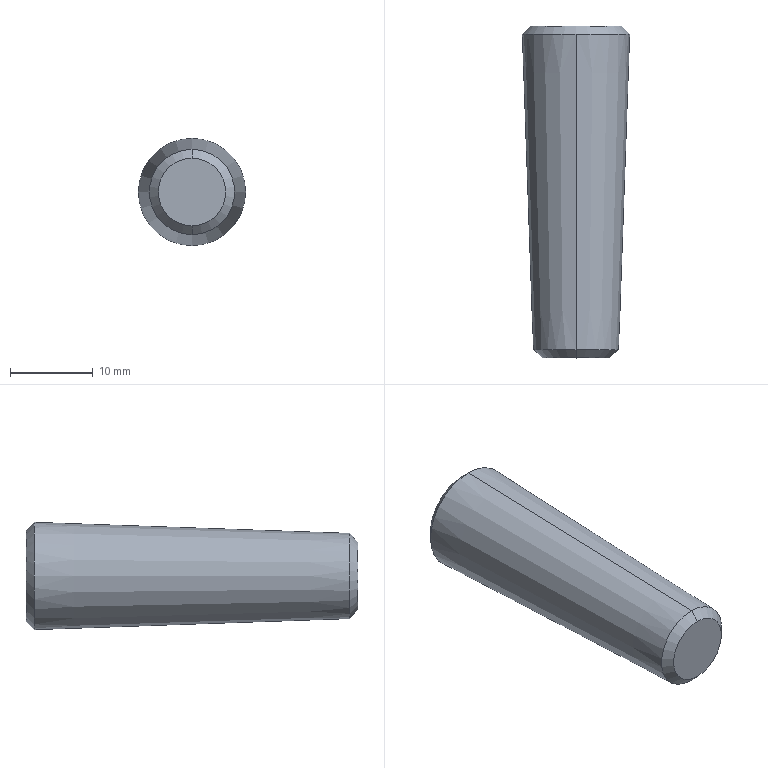Component | SolidWorks | TaperPin-1 | 1 solid | 8 faces | box 12.93 x 40 x 12.93 mm | volume 4216 mm3 | cone 6 | plane 2
build123d program:
from build123d import *
from OCP.BRepFilletAPI import BRepFilletAPI_MakeChamfer

# Parameters (mm, degrees)
CHAMFER1_SIZE    = 1
CHAMFER1_SIZE2   = 1.037
CHAMFER1_SIZE2_2 = 0.9668


with BuildPart() as part:
    # Sketch1 → Revolve4 (revolve)
    with BuildSketch(Plane.XY, mode=Mode.PRIVATE) as revolve4_sk:
        Polygon((6.5, 40), (5.103, 0), (0, 0), (0, 40), align=None)
    revolve(revolve4_sk.sketch.rotate(Axis((0, 0, 0), (0, 1, 0)), 90), axis=Axis((0, 0, 0), (0, 1, 0)))

    # Chamfer1: one chamfer whose edges measure the first distance from different faces: ONE call of the kernel's chamfer builder (chamfer() names one face for all edges)
    chamfer1_edges_1 = [part.edges().sort_by_distance(p)[0] for p in [
        (0, 0, 5.103),
    ]]
    chamfer1_side_1 = [part.faces().sort_by_distance(p)[0] for p in [
        (0, 20, 5.802),
    ]]
    chamfer1_edges_2 = [part.edges().sort_by_distance(p)[0] for p in [
        (0, 40, 6.5),
    ]]
    chamfer1_side_2 = [part.faces().sort_by_distance(p)[0] for p in [
        (0, 40, 0),
    ]]
    chamfer1 = BRepFilletAPI_MakeChamfer(part.part.solid().wrapped)
    for e in chamfer1_edges_1:
        chamfer1.Add(CHAMFER1_SIZE, CHAMFER1_SIZE2, e.wrapped, chamfer1_side_1[0].wrapped)  # the first distance lies on this face
    for e in chamfer1_edges_2:
        chamfer1.Add(CHAMFER1_SIZE, CHAMFER1_SIZE2_2, e.wrapped, chamfer1_side_2[0].wrapped)  # the first distance lies on this face
    add(Compound.cast(chamfer1.Shape()), mode=Mode.REPLACE)


solid = part.part

# Placed as in the assembly
solid = solid.moved(Location((726.83, 1259.341, 1507.217), (0, 0, 0)))
STEP:
#1=COLOUR_RGB('',0.7922,0.8196,0.9333);
#2=FILL_AREA_STYLE_COLOUR('',#1);
#3=FILL_AREA_STYLE('',(#2));
#4=SURFACE_STYLE_FILL_AREA(#3);
#5=SURFACE_SIDE_STYLE('',(#4));
#6=SURFACE_STYLE_USAGE(.BOTH.,#5);
#7=PRESENTATION_STYLE_ASSIGNMENT((#6));
#8=CARTESIAN_POINT('',(28.615,51.155,59.556));
#9=VERTEX_POINT('',#8);
#10=CARTESIAN_POINT('',(28.615,51.155,59.123));
#11=VERTEX_POINT('',#10);
#12=CARTESIAN_POINT('',(28.615,51.155,59.339));
#13=DIRECTION('',(0.,1.,0.));
#14=DIRECTION('',(0.,0.,-1.));
#15=AXIS2_PLACEMENT_3D('',#12,#13,#14);
#16=CIRCLE('',#15,0.2165);
#17=EDGE_CURVE('',#9,#11,#16,.T.);
#18=ORIENTED_EDGE('',*,*,#17,.F.);
#19=CARTESIAN_POINT('',(28.615,51.117,59.594));
#20=VERTEX_POINT('',#19);
#21=CARTESIAN_POINT('',(28.615,51.117,59.594));
#22=DIRECTION('',(0.,-0.7071,0.7071));
#23=VECTOR('',#22,39.37);
#24=LINE('',#21,#23);
#25=EDGE_CURVE('',#9,#20,#24,.T.);
#26=ORIENTED_EDGE('',*,*,#25,.T.);
#27=CARTESIAN_POINT('',(28.615,51.117,59.085));
#28=VERTEX_POINT('',#27);
#29=CARTESIAN_POINT('',(28.615,51.117,59.339));
#30=DIRECTION('',(0.,-1.,0.));
#31=DIRECTION('',(0.,0.,-1.));
#32=AXIS2_PLACEMENT_3D('',#29,#30,#31);
#33=CIRCLE('',#32,0.2546);
#34=EDGE_CURVE('',#28,#20,#33,.T.);
#35=ORIENTED_EDGE('',*,*,#34,.F.);
#36=CARTESIAN_POINT('',(28.615,51.117,59.085));
#37=DIRECTION('',(0.,-0.7071,-0.7071));
#38=VECTOR('',#37,39.37);
#39=LINE('',#36,#38);
#40=EDGE_CURVE('',#11,#28,#39,.T.);
#41=ORIENTED_EDGE('',*,*,#40,.F.);
#42=EDGE_LOOP('',(#18,#26,#35,#41));
#43=FACE_OUTER_BOUND('',#42,.T.);
#44=CARTESIAN_POINT('',(28.615,51.117,59.339));
#45=DIRECTION('',(0.,-1.,0.));
#46=DIRECTION('',(0.,0.,-1.));
#47=AXIS2_PLACEMENT_3D('',#44,#45,#46);
#48=CONICAL_SURFACE('',#47,0.2546,0.7854);
#49=ADVANCED_FACE('',(#43),#48,.T.);
#50=CARTESIAN_POINT('',(28.615,49.58,59.179));
#51=VERTEX_POINT('',#50);
#52=CARTESIAN_POINT('',(28.615,49.58,59.499));
#53=VERTEX_POINT('',#52);
#54=CARTESIAN_POINT('',(28.615,49.58,59.339));
#55=DIRECTION('',(0.,-1.,0.));
#56=DIRECTION('',(0.,0.,-1.));
#57=AXIS2_PLACEMENT_3D('',#54,#55,#56);
#58=CIRCLE('',#57,0.1601);
#59=EDGE_CURVE('',#51,#53,#58,.T.);
#60=ORIENTED_EDGE('',*,*,#59,.F.);
#61=CARTESIAN_POINT('',(28.615,49.62,59.137));
#62=VERTEX_POINT('',#61);
#63=CARTESIAN_POINT('',(28.615,49.58,59.179));
#64=DIRECTION('',(0.,0.682,-0.7314));
#65=VECTOR('',#64,39.37);
#66=LINE('',#63,#65);
#67=EDGE_CURVE('',#51,#62,#66,.T.);
#68=ORIENTED_EDGE('',*,*,#67,.T.);
#69=CARTESIAN_POINT('',(28.615,49.62,59.542));
#70=VERTEX_POINT('',#69);
#71=CARTESIAN_POINT('',(28.615,49.62,59.339));
#72=DIRECTION('',(0.,1.,0.));
#73=DIRECTION('',(0.,0.,1.));
#74=AXIS2_PLACEMENT_3D('',#71,#72,#73);
#75=CIRCLE('',#74,0.2023);
#76=EDGE_CURVE('',#70,#62,#75,.T.);
#77=ORIENTED_EDGE('',*,*,#76,.F.);
#78=CARTESIAN_POINT('',(28.615,49.58,59.499));
#79=DIRECTION('',(0.,0.682,0.7314));
#80=VECTOR('',#79,39.37);
#81=LINE('',#78,#80);
#82=EDGE_CURVE('',#53,#70,#81,.T.);
#83=ORIENTED_EDGE('',*,*,#82,.F.);
#84=EDGE_LOOP('',(#60,#68,#77,#83));
#85=FACE_OUTER_BOUND('',#84,.T.);
#86=CARTESIAN_POINT('',(28.615,49.58,59.339));
#87=DIRECTION('',(0.,1.,0.));
#88=DIRECTION('',(0.,0.,1.));
#89=AXIS2_PLACEMENT_3D('',#86,#87,#88);
#90=CONICAL_SURFACE('',#89,0.1601,0.8203);
#91=ADVANCED_FACE('',(#85),#90,.T.);
#92=ORIENTED_EDGE('',*,*,#76,.T.);
#93=CARTESIAN_POINT('',(28.615,51.155,59.083));
#94=DIRECTION('',(0.,0.9994,-0.0349));
#95=VECTOR('',#94,39.37);
#96=LINE('',#93,#95);
#97=EDGE_CURVE('',#62,#28,#96,.T.);
#98=ORIENTED_EDGE('',*,*,#97,.T.);
#99=ORIENTED_EDGE('',*,*,#34,.T.);
#100=CARTESIAN_POINT('',(28.615,51.155,59.595));
#101=DIRECTION('',(0.,0.9994,0.0349));
#102=VECTOR('',#101,39.37);
#103=LINE('',#100,#102);
#104=EDGE_CURVE('',#70,#20,#103,.T.);
#105=ORIENTED_EDGE('',*,*,#104,.F.);
#106=EDGE_LOOP('',(#92,#98,#99,#105));
#107=FACE_OUTER_BOUND('',#106,.T.);
#108=CARTESIAN_POINT('',(28.615,51.155,59.339));
#109=DIRECTION('',(0.,1.,0.));
#110=DIRECTION('',(0.,0.,1.));
#111=AXIS2_PLACEMENT_3D('',#108,#109,#110);
#112=CONICAL_SURFACE('',#111,0.2559,0.03491);
#113=ADVANCED_FACE('',(#107),#112,.T.);
#114=ORIENTED_EDGE('',*,*,#97,.F.);
#115=CARTESIAN_POINT('',(28.615,49.62,59.339));
#116=DIRECTION('',(0.,1.,0.));
#117=DIRECTION('',(0.,0.,1.));
#118=AXIS2_PLACEMENT_3D('',#115,#116,#117);
#119=CIRCLE('',#118,0.2023);
#120=EDGE_CURVE('',#62,#70,#119,.T.);
#121=ORIENTED_EDGE('',*,*,#120,.T.);
#122=ORIENTED_EDGE('',*,*,#104,.T.);
#123=CARTESIAN_POINT('',(28.615,51.117,59.339));
#124=DIRECTION('',(0.,-1.,0.));
#125=DIRECTION('',(0.,0.,-1.));
#126=AXIS2_PLACEMENT_3D('',#123,#124,#125);
#127=CIRCLE('',#126,0.2546);
#128=EDGE_CURVE('',#20,#28,#127,.T.);
#129=ORIENTED_EDGE('',*,*,#128,.T.);
#130=EDGE_LOOP('',(#114,#121,#122,#129));
#131=FACE_OUTER_BOUND('',#130,.T.);
#132=CARTESIAN_POINT('',(28.615,51.155,59.339));
#133=DIRECTION('',(0.,1.,0.));
#134=DIRECTION('',(0.,0.,1.));
#135=AXIS2_PLACEMENT_3D('',#132,#133,#134);
#136=CONICAL_SURFACE('',#135,0.2559,0.03491);
#137=ADVANCED_FACE('',(#131),#136,.T.);
#138=CARTESIAN_POINT('',(28.615,51.155,59.339));
#139=DIRECTION('',(0.,1.,0.));
#140=DIRECTION('',(0.,0.,-1.));
#141=AXIS2_PLACEMENT_3D('',#138,#139,#140);
#142=CIRCLE('',#141,0.2165);
#143=EDGE_CURVE('',#11,#9,#142,.T.);
#144=ORIENTED_EDGE('',*,*,#143,.T.);
#145=ORIENTED_EDGE('',*,*,#17,.T.);
#146=EDGE_LOOP('',(#144,#145));
#147=FACE_OUTER_BOUND('',#146,.T.);
#148=CARTESIAN_POINT('',(28.615,51.155,59.339));
#149=DIRECTION('',(0.,-1.,0.));
#150=DIRECTION('',(0.,0.,-1.));
#151=AXIS2_PLACEMENT_3D('',#148,#149,#150);
#152=PLANE('',#151);
#153=ADVANCED_FACE('',(#147),#152,.F.);
#154=CARTESIAN_POINT('',(28.615,49.58,59.339));
#155=DIRECTION('',(0.,-1.,0.));
#156=DIRECTION('',(0.,0.,-1.));
#157=AXIS2_PLACEMENT_3D('',#154,#155,#156);
#158=CIRCLE('',#157,0.1601);
#159=EDGE_CURVE('',#53,#51,#158,.T.);
#160=ORIENTED_EDGE('',*,*,#159,.T.);
#161=ORIENTED_EDGE('',*,*,#59,.T.);
#162=EDGE_LOOP('',(#160,#161));
#163=FACE_OUTER_BOUND('',#162,.T.);
#164=CARTESIAN_POINT('',(28.615,49.58,59.339));
#165=DIRECTION('',(0.,-1.,0.));
#166=DIRECTION('',(0.,0.,-1.));
#167=AXIS2_PLACEMENT_3D('',#164,#165,#166);
#168=PLANE('',#167);
#169=ADVANCED_FACE('',(#163),#168,.T.);
#170=ORIENTED_EDGE('',*,*,#67,.F.);
#171=ORIENTED_EDGE('',*,*,#159,.F.);
#172=ORIENTED_EDGE('',*,*,#82,.T.);
#173=ORIENTED_EDGE('',*,*,#120,.F.);
#174=EDGE_LOOP('',(#170,#171,#172,#173));
#175=FACE_OUTER_BOUND('',#174,.T.);
#176=CARTESIAN_POINT('',(28.615,49.58,59.339));
#177=DIRECTION('',(0.,1.,0.));
#178=DIRECTION('',(0.,0.,1.));
#179=AXIS2_PLACEMENT_3D('',#176,#177,#178);
#180=CONICAL_SURFACE('',#179,0.1601,0.8203);
#181=ADVANCED_FACE('',(#175),#180,.T.);
#182=ORIENTED_EDGE('',*,*,#25,.F.);
#183=ORIENTED_EDGE('',*,*,#143,.F.);
#184=ORIENTED_EDGE('',*,*,#40,.T.);
#185=ORIENTED_EDGE('',*,*,#128,.F.);
#186=EDGE_LOOP('',(#182,#183,#184,#185));
#187=FACE_OUTER_BOUND('',#186,.T.);
#188=CARTESIAN_POINT('',(28.615,51.117,59.339));
#189=DIRECTION('',(0.,-1.,0.));
#190=DIRECTION('',(0.,0.,-1.));
#191=AXIS2_PLACEMENT_3D('',#188,#189,#190);
#192=CONICAL_SURFACE('',#191,0.2546,0.7854);
#193=ADVANCED_FACE('',(#187),#192,.T.);
#194=CLOSED_SHELL('',(#49,#91,#113,#137,#153,#169,#181,#193));
#195=MANIFOLD_SOLID_BREP('',#194);
#196=STYLED_ITEM('',(#7),#195);
#197=PRESENTATION_LAYER_ASSIGNMENT('','',(#196));
#198=CARTESIAN_POINT('',(0.,0.,0.));
#199=DIRECTION('',(0.,0.,1.));
#200=DIRECTION('',(1.,0.,0.));
#201=AXIS2_PLACEMENT_3D('',#198,#199,#200);
#202=(LENGTH_UNIT()NAMED_UNIT(*)SI_UNIT($,.METRE.));
#203=LENGTH_MEASURE_WITH_UNIT(LENGTH_MEASURE(0.0254),#202);
#204=DIMENSIONAL_EXPONENTS(1.,0.,0.,0.,0.,0.,0.);
#205=(CONVERSION_BASED_UNIT('',#203)LENGTH_UNIT()NAMED_UNIT(#204));
#206=UNCERTAINTY_MEASURE_WITH_UNIT(LENGTH_MEASURE(0.00001),#205,'','');
#207=(NAMED_UNIT(*)PLANE_ANGLE_UNIT()SI_UNIT($,.RADIAN.));
#208=(NAMED_UNIT(*)SI_UNIT($,.STERADIAN.)SOLID_ANGLE_UNIT());
#209=(GEOMETRIC_REPRESENTATION_CONTEXT(3)GLOBAL_UNCERTAINTY_ASSIGNED_CONTEXT((#206))GLOBAL_UNIT_ASSIGNED_CONTEXT((#205,#207,#208))REPRESENTATION_CONTEXT('',''));
#210=ADVANCED_BREP_SHAPE_REPRESENTATION('',(#195,#201),#209);
#211=(LENGTH_UNIT()NAMED_UNIT(*)SI_UNIT($,.METRE.));
#212=LENGTH_MEASURE_WITH_UNIT(LENGTH_MEASURE(0.0254),#211);
#213=DIMENSIONAL_EXPONENTS(1.,0.,0.,0.,0.,0.,0.);
#214=(CONVERSION_BASED_UNIT('',#212)LENGTH_UNIT()NAMED_UNIT(#213));
#215=UNCERTAINTY_MEASURE_WITH_UNIT(LENGTH_MEASURE(0.00001),#214,'','');
#216=(NAMED_UNIT(*)PLANE_ANGLE_UNIT()SI_UNIT($,.RADIAN.));
#217=(NAMED_UNIT(*)SI_UNIT($,.STERADIAN.)SOLID_ANGLE_UNIT());
#218=(GEOMETRIC_REPRESENTATION_CONTEXT(3)GLOBAL_UNCERTAINTY_ASSIGNED_CONTEXT((#215))GLOBAL_UNIT_ASSIGNED_CONTEXT((#214,#216,#217))REPRESENTATION_CONTEXT('',''));
#219=MECHANICAL_DESIGN_GEOMETRIC_PRESENTATION_REPRESENTATION('',(#196),#218);